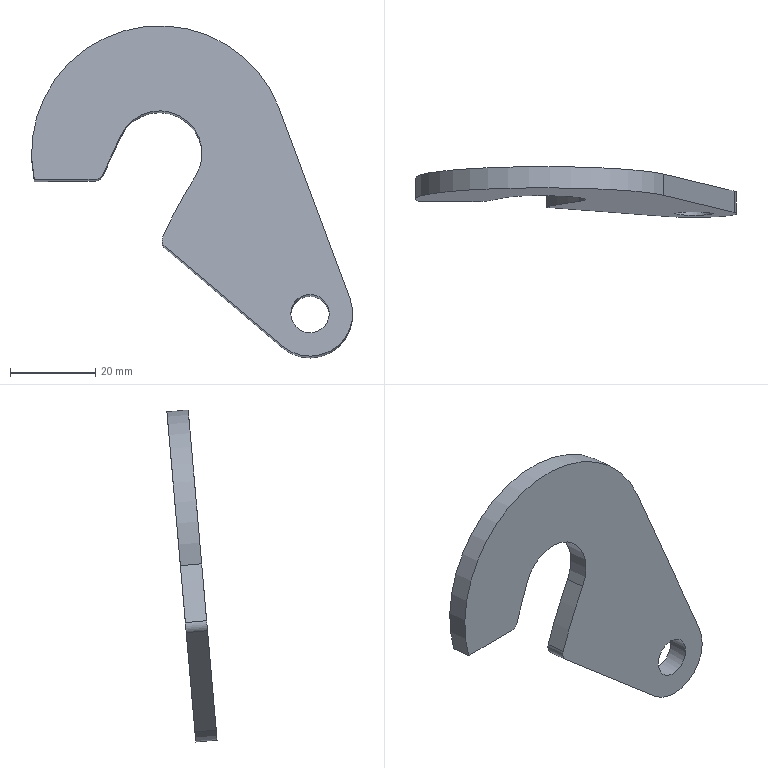Component | NX | HOOK_BAFFLE | 1 solid | 13 faces | box 75.29 x 11.76 x 77.87 mm | volume 13326 mm3 | cylinder 7 | plane 6 | commonest cylinder face diameters 20 x2 4 x2 60 x1 254.505 x1 9 x1
STEP:
#1=CARTESIAN_POINT('',(0.,0.,0.));
#2=DIRECTION('',(0.,0.,1.));
#3=DIRECTION('',(1.,0.,0.));
#4=AXIS2_PLACEMENT_3D('',#1,#2,#3);
#5=CARTESIAN_POINT('',(364.754,540.035,-52.402));
#6=VERTEX_POINT('',#5);
#7=CARTESIAN_POINT('',(380.609,541.002,-41.353));
#8=VERTEX_POINT('',#7);
#9=CARTESIAN_POINT('',(371.23,540.7,-44.811));
#10=DIRECTION('',(0.,-0.9962,0.08716));
#11=DIRECTION('',(-1.,-0.0006658,-0.00761));
#12=AXIS2_PLACEMENT_3D('',#9,#10,#11);
#13=CIRCLE('',#12,10.);
#14=CARTESIAN_POINT('',(371.23,545.681,-45.247));
#15=DIRECTION('',(0.,-0.9962,0.08716));
#16=DIRECTION('',(-0.00764,0.08715,0.9962));
#17=AXIS2_PLACEMENT_3D('',#14,#15,#16);
#18=CYLINDRICAL_SURFACE('',#17,10.);
#19=CARTESIAN_POINT('',(1.571,5.));
#20=DIRECTION('',(1.,-0.));
#21=VECTOR('',#20,1.);
#22=LINE('',#19,#21);
#23=(GEOMETRIC_REPRESENTATION_CONTEXT(2)PARAMETRIC_REPRESENTATION_CONTEXT()REPRESENTATION_CONTEXT('',''));
#24=DEFINITIONAL_REPRESENTATION('',(#22),#23);
#25=PCURVE('',#18,#24);
#26=CARTESIAN_POINT('',(371.23,540.7,-44.811));
#27=DIRECTION('',(0.,-0.9962,0.08716));
#28=DIRECTION('',(-0.00764,0.08715,0.9962));
#29=AXIS2_PLACEMENT_3D('',#26,#27,#28);
#30=PLANE('',#29);
#31=CARTESIAN_POINT('',(0.,0.));
#32=DIRECTION('',(0.,1.));
#33=AXIS2_PLACEMENT_2D('',#31,#32);
#34=CIRCLE('',#33,10.);
#35=(GEOMETRIC_REPRESENTATION_CONTEXT(2)PARAMETRIC_REPRESENTATION_CONTEXT()REPRESENTATION_CONTEXT('',''));
#36=DEFINITIONAL_REPRESENTATION('',(#34),#35);
#37=PCURVE('',#30,#36);
#38=SURFACE_CURVE('',#13,(#25,#37),.PCURVE_S1.);
#39=EDGE_CURVE('',#6,#8,#38,.T.);
#40=ORIENTED_EDGE('',*,*,#39,.F.);
#41=CARTESIAN_POINT('',(364.754,545.016,-52.838));
#42=VERTEX_POINT('',#41);
#43=CARTESIAN_POINT('',(364.754,545.016,-52.838));
#44=DIRECTION('',(0.,-0.9962,0.08716));
#45=VECTOR('',#44,1.);
#46=LINE('',#43,#45);
#47=CARTESIAN_POINT('',(2.43,-0.));
#48=DIRECTION('',(0.,1.));
#49=VECTOR('',#48,1.);
#50=LINE('',#47,#49);
#51=(GEOMETRIC_REPRESENTATION_CONTEXT(2)PARAMETRIC_REPRESENTATION_CONTEXT()REPRESENTATION_CONTEXT('',''));
#52=DEFINITIONAL_REPRESENTATION('',(#50),#51);
#53=PCURVE('',#18,#52);
#54=CARTESIAN_POINT('',(336.102,547.139,-28.578));
#55=DIRECTION('',(-0.6476,-0.06641,-0.7591));
#56=DIRECTION('',(-0.762,0.05644,0.6451));
#57=AXIS2_PLACEMENT_3D('',#54,#55,#56);
#58=PLANE('',#57);
#59=CARTESIAN_POINT('',(-37.603,0.));
#60=DIRECTION('',(0.,-1.));
#61=VECTOR('',#60,1.);
#62=LINE('',#59,#61);
#63=(GEOMETRIC_REPRESENTATION_CONTEXT(2)PARAMETRIC_REPRESENTATION_CONTEXT()REPRESENTATION_CONTEXT('',''));
#64=DEFINITIONAL_REPRESENTATION('',(#62),#63);
#65=PCURVE('',#58,#64);
#66=SURFACE_CURVE('',#46,(#53,#65),.PCURVE_S1.);
#67=EDGE_CURVE('',#42,#6,#66,.T.);
#68=ORIENTED_EDGE('',*,*,#67,.F.);
#69=CARTESIAN_POINT('',(380.609,545.983,-41.789));
#70=VERTEX_POINT('',#69);
#71=CARTESIAN_POINT('',(371.23,545.681,-45.247));
#72=DIRECTION('',(0.,-0.9962,0.08716));
#73=DIRECTION('',(-1.,-0.0006658,-0.00761));
#74=AXIS2_PLACEMENT_3D('',#71,#72,#73);
#75=CIRCLE('',#74,10.);
#76=CARTESIAN_POINT('',(1.571,0.));
#77=DIRECTION('',(1.,-0.));
#78=VECTOR('',#77,1.);
#79=LINE('',#76,#78);
#80=(GEOMETRIC_REPRESENTATION_CONTEXT(2)PARAMETRIC_REPRESENTATION_CONTEXT()REPRESENTATION_CONTEXT('',''));
#81=DEFINITIONAL_REPRESENTATION('',(#79),#80);
#82=PCURVE('',#18,#81);
#83=CARTESIAN_POINT('',(371.23,545.681,-45.247));
#84=DIRECTION('',(0.,-0.9962,0.08716));
#85=DIRECTION('',(-0.00764,0.08715,0.9962));
#86=AXIS2_PLACEMENT_3D('',#83,#84,#85);
#87=PLANE('',#86);
#88=CARTESIAN_POINT('',(0.,0.));
#89=DIRECTION('',(0.,1.));
#90=AXIS2_PLACEMENT_2D('',#88,#89);
#91=CIRCLE('',#90,10.);
#92=(GEOMETRIC_REPRESENTATION_CONTEXT(2)PARAMETRIC_REPRESENTATION_CONTEXT()REPRESENTATION_CONTEXT('',''));
#93=DEFINITIONAL_REPRESENTATION('',(#91),#92);
#94=PCURVE('',#87,#93);
#95=SURFACE_CURVE('',#75,(#82,#94),.PCURVE_S1.);
#96=EDGE_CURVE('',#42,#70,#95,.T.);
#97=ORIENTED_EDGE('',*,*,#96,.T.);
#98=CARTESIAN_POINT('',(380.609,545.983,-41.789));
#99=DIRECTION('',(0.,-0.9962,0.08716));
#100=VECTOR('',#99,1.);
#101=LINE('',#98,#100);
#102=CARTESIAN_POINT('',(5.059,-0.));
#103=DIRECTION('',(-0.,1.));
#104=VECTOR('',#103,1.);
#105=LINE('',#102,#104);
#106=(GEOMETRIC_REPRESENTATION_CONTEXT(2)PARAMETRIC_REPRESENTATION_CONTEXT()REPRESENTATION_CONTEXT('',''));
#107=DEFINITIONAL_REPRESENTATION('',(#105),#106);
#108=PCURVE('',#18,#107);
#109=CARTESIAN_POINT('',(380.609,545.983,-41.789));
#110=DIRECTION('',(0.9378,0.03025,0.3458));
#111=DIRECTION('',(0.3471,-0.08174,-0.9343));
#112=AXIS2_PLACEMENT_3D('',#109,#110,#111);
#113=PLANE('',#112);
#114=CARTESIAN_POINT('',(-0.,-0.));
#115=DIRECTION('',(-0.,-1.));
#116=VECTOR('',#115,1.);
#117=LINE('',#114,#116);
#118=(GEOMETRIC_REPRESENTATION_CONTEXT(2)PARAMETRIC_REPRESENTATION_CONTEXT()REPRESENTATION_CONTEXT('',''));
#119=DEFINITIONAL_REPRESENTATION('',(#117),#118);
#120=PCURVE('',#113,#119);
#121=SURFACE_CURVE('',#101,(#108,#120),.PCURVE_S1.);
#122=EDGE_CURVE('',#70,#8,#121,.T.);
#123=ORIENTED_EDGE('',*,*,#122,.T.);
#124=EDGE_LOOP('',(#40,#68,#97,#123));
#125=FACE_BOUND('',#124,.T.);
#126=ADVANCED_FACE('',(#125),#18,.T.);
#127=CARTESIAN_POINT('',(364.076,544.896,3.15));
#128=VERTEX_POINT('',#127);
#129=CARTESIAN_POINT('',(380.609,541.002,-41.353));
#130=DIRECTION('',(-0.3471,0.08174,0.9343));
#131=VECTOR('',#130,1.);
#132=LINE('',#129,#131);
#133=CARTESIAN_POINT('',(0.,-5.));
#134=DIRECTION('',(-1.,0.));
#135=VECTOR('',#134,1.);
#136=LINE('',#133,#135);
#137=(GEOMETRIC_REPRESENTATION_CONTEXT(2)PARAMETRIC_REPRESENTATION_CONTEXT()REPRESENTATION_CONTEXT('',''));
#138=DEFINITIONAL_REPRESENTATION('',(#136),#137);
#139=PCURVE('',#113,#138);
#140=CARTESIAN_POINT('',(3.399,-9.405));
#141=DIRECTION('',(0.9405,0.3399));
#142=VECTOR('',#141,1.);
#143=LINE('',#140,#142);
#144=(GEOMETRIC_REPRESENTATION_CONTEXT(2)PARAMETRIC_REPRESENTATION_CONTEXT()REPRESENTATION_CONTEXT('',''));
#145=DEFINITIONAL_REPRESENTATION('',(#143),#144);
#146=PCURVE('',#30,#145);
#147=SURFACE_CURVE('',#132,(#139,#146),.PCURVE_S1.);
#148=EDGE_CURVE('',#8,#128,#147,.T.);
#149=ORIENTED_EDGE('',*,*,#148,.F.);
#150=ORIENTED_EDGE('',*,*,#122,.F.);
#151=CARTESIAN_POINT('',(364.076,549.877,2.714));
#152=VERTEX_POINT('',#151);
#153=CARTESIAN_POINT('',(380.609,545.983,-41.789));
#154=DIRECTION('',(-0.3471,0.08174,0.9343));
#155=VECTOR('',#154,1.);
#156=LINE('',#153,#155);
#157=CARTESIAN_POINT('',(0.,0.));
#158=DIRECTION('',(-1.,0.));
#159=VECTOR('',#158,1.);
#160=LINE('',#157,#159);
#161=(GEOMETRIC_REPRESENTATION_CONTEXT(2)PARAMETRIC_REPRESENTATION_CONTEXT()REPRESENTATION_CONTEXT('',''));
#162=DEFINITIONAL_REPRESENTATION('',(#160),#161);
#163=PCURVE('',#113,#162);
#164=CARTESIAN_POINT('',(3.399,-9.405));
#165=DIRECTION('',(0.9405,0.3399));
#166=VECTOR('',#165,1.);
#167=LINE('',#164,#166);
#168=(GEOMETRIC_REPRESENTATION_CONTEXT(2)PARAMETRIC_REPRESENTATION_CONTEXT()REPRESENTATION_CONTEXT('',''));
#169=DEFINITIONAL_REPRESENTATION('',(#167),#168);
#170=PCURVE('',#87,#169);
#171=SURFACE_CURVE('',#156,(#163,#170),.PCURVE_S1.);
#172=EDGE_CURVE('',#70,#152,#171,.T.);
#173=ORIENTED_EDGE('',*,*,#172,.T.);
#174=CARTESIAN_POINT('',(364.076,549.877,2.714));
#175=DIRECTION('',(0.,-0.9962,0.08716));
#176=VECTOR('',#175,1.);
#177=LINE('',#174,#176);
#178=CARTESIAN_POINT('',(-47.634,0.));
#179=DIRECTION('',(-0.,-1.));
#180=VECTOR('',#179,1.);
#181=LINE('',#178,#180);
#182=(GEOMETRIC_REPRESENTATION_CONTEXT(2)PARAMETRIC_REPRESENTATION_CONTEXT()REPRESENTATION_CONTEXT('',''));
#183=DEFINITIONAL_REPRESENTATION('',(#181),#182);
#184=PCURVE('',#113,#183);
#185=CARTESIAN_POINT('',(335.941,548.969,-7.659));
#186=DIRECTION('',(0.,-0.9962,0.08716));
#187=DIRECTION('',(-0.00764,0.08715,0.9962));
#188=AXIS2_PLACEMENT_3D('',#185,#186,#187);
#189=CYLINDRICAL_SURFACE('',#188,30.);
#190=CARTESIAN_POINT('',(-1.224,-0.));
#191=DIRECTION('',(0.,1.));
#192=VECTOR('',#191,1.);
#193=LINE('',#190,#192);
#194=(GEOMETRIC_REPRESENTATION_CONTEXT(2)PARAMETRIC_REPRESENTATION_CONTEXT()REPRESENTATION_CONTEXT('',''));
#195=DEFINITIONAL_REPRESENTATION('',(#193),#194);
#196=PCURVE('',#189,#195);
#197=SURFACE_CURVE('',#177,(#184,#196),.PCURVE_S1.);
#198=EDGE_CURVE('',#152,#128,#197,.T.);
#199=ORIENTED_EDGE('',*,*,#198,.T.);
#200=EDGE_LOOP('',(#149,#150,#173,#199));
#201=FACE_BOUND('',#200,.T.);
#202=ADVANCED_FACE('',(#201),#113,.T.);
#203=CARTESIAN_POINT('',(306.594,543.446,-13.424));
#204=VERTEX_POINT('',#203);
#205=CARTESIAN_POINT('',(335.941,543.988,-7.223));
#206=DIRECTION('',(0.,-0.9962,0.08716));
#207=DIRECTION('',(-1.,-0.0006658,-0.00761));
#208=AXIS2_PLACEMENT_3D('',#205,#206,#207);
#209=CIRCLE('',#208,30.);
#210=CARTESIAN_POINT('',(-4.712,5.));
#211=DIRECTION('',(1.,0.));
#212=VECTOR('',#211,1.);
#213=LINE('',#210,#212);
#214=(GEOMETRIC_REPRESENTATION_CONTEXT(2)PARAMETRIC_REPRESENTATION_CONTEXT()REPRESENTATION_CONTEXT('',''));
#215=DEFINITIONAL_REPRESENTATION('',(#213),#214);
#216=PCURVE('',#189,#215);
#217=CARTESIAN_POINT('',(38.,35.));
#218=DIRECTION('',(0.,1.));
#219=AXIS2_PLACEMENT_2D('',#217,#218);
#220=CIRCLE('',#219,30.);
#221=(GEOMETRIC_REPRESENTATION_CONTEXT(2)PARAMETRIC_REPRESENTATION_CONTEXT()REPRESENTATION_CONTEXT('',''));
#222=DEFINITIONAL_REPRESENTATION('',(#220),#221);
#223=PCURVE('',#30,#222);
#224=SURFACE_CURVE('',#209,(#216,#223),.PCURVE_S1.);
#225=EDGE_CURVE('',#128,#204,#224,.T.);
#226=ORIENTED_EDGE('',*,*,#225,.F.);
#227=ORIENTED_EDGE('',*,*,#198,.F.);
#228=CARTESIAN_POINT('',(306.594,548.427,-13.86));
#229=VERTEX_POINT('',#228);
#230=CARTESIAN_POINT('',(335.941,548.969,-7.659));
#231=DIRECTION('',(0.,-0.9962,0.08716));
#232=DIRECTION('',(-1.,-0.0006658,-0.00761));
#233=AXIS2_PLACEMENT_3D('',#230,#231,#232);
#234=CIRCLE('',#233,30.);
#235=CARTESIAN_POINT('',(-4.712,0.));
#236=DIRECTION('',(1.,-0.));
#237=VECTOR('',#236,1.);
#238=LINE('',#235,#237);
#239=(GEOMETRIC_REPRESENTATION_CONTEXT(2)PARAMETRIC_REPRESENTATION_CONTEXT()REPRESENTATION_CONTEXT('',''));
#240=DEFINITIONAL_REPRESENTATION('',(#238),#239);
#241=PCURVE('',#189,#240);
#242=CARTESIAN_POINT('',(38.,35.));
#243=DIRECTION('',(0.,1.));
#244=AXIS2_PLACEMENT_2D('',#242,#243);
#245=CIRCLE('',#244,30.);
#246=(GEOMETRIC_REPRESENTATION_CONTEXT(2)PARAMETRIC_REPRESENTATION_CONTEXT()REPRESENTATION_CONTEXT('',''));
#247=DEFINITIONAL_REPRESENTATION('',(#245),#246);
#248=PCURVE('',#87,#247);
#249=SURFACE_CURVE('',#234,(#241,#248),.PCURVE_S1.);
#250=EDGE_CURVE('',#152,#229,#249,.T.);
#251=ORIENTED_EDGE('',*,*,#250,.T.);
#252=CARTESIAN_POINT('',(306.594,548.427,-13.86));
#253=DIRECTION('',(0.,-0.9962,0.08716));
#254=VECTOR('',#253,1.);
#255=LINE('',#252,#254);
#256=CARTESIAN_POINT('',(1.772,-0.));
#257=DIRECTION('',(0.,1.));
#258=VECTOR('',#257,1.);
#259=LINE('',#256,#258);
#260=(GEOMETRIC_REPRESENTATION_CONTEXT(2)PARAMETRIC_REPRESENTATION_CONTEXT()REPRESENTATION_CONTEXT('',''));
#261=DEFINITIONAL_REPRESENTATION('',(#259),#260);
#262=PCURVE('',#189,#261);
#263=CARTESIAN_POINT('',(306.594,548.427,-13.86));
#264=DIRECTION('',(0.00764,-0.08715,-0.9962));
#265=DIRECTION('',(-0.,-0.9962,0.08716));
#266=AXIS2_PLACEMENT_3D('',#263,#264,#265);
#267=PLANE('',#266);
#268=CARTESIAN_POINT('',(0.,0.));
#269=DIRECTION('',(1.,0.));
#270=VECTOR('',#269,1.);
#271=LINE('',#268,#270);
#272=(GEOMETRIC_REPRESENTATION_CONTEXT(2)PARAMETRIC_REPRESENTATION_CONTEXT()REPRESENTATION_CONTEXT('',''));
#273=DEFINITIONAL_REPRESENTATION('',(#271),#272);
#274=PCURVE('',#267,#273);
#275=SURFACE_CURVE('',#255,(#262,#274),.PCURVE_S1.);
#276=EDGE_CURVE('',#229,#204,#275,.T.);
#277=ORIENTED_EDGE('',*,*,#276,.T.);
#278=EDGE_LOOP('',(#226,#227,#251,#277));
#279=FACE_BOUND('',#278,.T.);
#280=ADVANCED_FACE('',(#279),#189,.T.);
#281=CARTESIAN_POINT('',(320.846,548.436,-13.751));
#282=VERTEX_POINT('',#281);
#283=CARTESIAN_POINT('',(306.594,548.427,-13.86));
#284=DIRECTION('',(1.,0.0006658,0.00761));
#285=VECTOR('',#284,1.);
#286=LINE('',#283,#285);
#287=CARTESIAN_POINT('',(0.,0.));
#288=DIRECTION('',(-0.,-1.));
#289=VECTOR('',#288,1.);
#290=LINE('',#287,#289);
#291=(GEOMETRIC_REPRESENTATION_CONTEXT(2)PARAMETRIC_REPRESENTATION_CONTEXT()REPRESENTATION_CONTEXT('',''));
#292=DEFINITIONAL_REPRESENTATION('',(#290),#291);
#293=PCURVE('',#267,#292);
#294=CARTESIAN_POINT('',(32.,64.394));
#295=DIRECTION('',(-0.,-1.));
#296=VECTOR('',#295,1.);
#297=LINE('',#294,#296);
#298=(GEOMETRIC_REPRESENTATION_CONTEXT(2)PARAMETRIC_REPRESENTATION_CONTEXT()REPRESENTATION_CONTEXT('',''));
#299=DEFINITIONAL_REPRESENTATION('',(#297),#298);
#300=PCURVE('',#87,#299);
#301=SURFACE_CURVE('',#286,(#293,#300),.PCURVE_S1.);
#302=EDGE_CURVE('',#229,#282,#301,.T.);
#303=ORIENTED_EDGE('',*,*,#302,.T.);
#304=CARTESIAN_POINT('',(320.846,543.455,-13.315));
#305=VERTEX_POINT('',#304);
#306=CARTESIAN_POINT('',(320.846,548.436,-13.751));
#307=DIRECTION('',(0.,-0.9962,0.08716));
#308=VECTOR('',#307,1.);
#309=LINE('',#306,#308);
#310=CARTESIAN_POINT('',(0.,-14.252));
#311=DIRECTION('',(1.,0.));
#312=VECTOR('',#311,1.);
#313=LINE('',#310,#312);
#314=(GEOMETRIC_REPRESENTATION_CONTEXT(2)PARAMETRIC_REPRESENTATION_CONTEXT()REPRESENTATION_CONTEXT('',''));
#315=DEFINITIONAL_REPRESENTATION('',(#313),#314);
#316=PCURVE('',#267,#315);
#317=CARTESIAN_POINT('',(320.83,548.61,-11.759));
#318=DIRECTION('',(0.,-0.9962,0.08716));
#319=DIRECTION('',(-0.00764,0.08715,0.9962));
#320=AXIS2_PLACEMENT_3D('',#317,#318,#319);
#321=CYLINDRICAL_SURFACE('',#320,2.);
#322=CARTESIAN_POINT('',(3.142,0.));
#323=DIRECTION('',(0.,1.));
#324=VECTOR('',#323,1.);
#325=LINE('',#322,#324);
#326=(GEOMETRIC_REPRESENTATION_CONTEXT(2)PARAMETRIC_REPRESENTATION_CONTEXT()REPRESENTATION_CONTEXT('',''));
#327=DEFINITIONAL_REPRESENTATION('',(#325),#326);
#328=PCURVE('',#321,#327);
#329=SURFACE_CURVE('',#309,(#316,#328),.PCURVE_S1.);
#330=EDGE_CURVE('',#282,#305,#329,.T.);
#331=ORIENTED_EDGE('',*,*,#330,.T.);
#332=CARTESIAN_POINT('',(306.594,543.446,-13.424));
#333=DIRECTION('',(1.,0.0006658,0.00761));
#334=VECTOR('',#333,1.);
#335=LINE('',#332,#334);
#336=CARTESIAN_POINT('',(5.,-0.));
#337=DIRECTION('',(-0.,-1.));
#338=VECTOR('',#337,1.);
#339=LINE('',#336,#338);
#340=(GEOMETRIC_REPRESENTATION_CONTEXT(2)PARAMETRIC_REPRESENTATION_CONTEXT()REPRESENTATION_CONTEXT('',''));
#341=DEFINITIONAL_REPRESENTATION('',(#339),#340);
#342=PCURVE('',#267,#341);
#343=CARTESIAN_POINT('',(32.,64.394));
#344=DIRECTION('',(-0.,-1.));
#345=VECTOR('',#344,1.);
#346=LINE('',#343,#345);
#347=(GEOMETRIC_REPRESENTATION_CONTEXT(2)PARAMETRIC_REPRESENTATION_CONTEXT()REPRESENTATION_CONTEXT('',''));
#348=DEFINITIONAL_REPRESENTATION('',(#346),#347);
#349=PCURVE('',#30,#348);
#350=SURFACE_CURVE('',#335,(#342,#349),.PCURVE_S1.);
#351=EDGE_CURVE('',#204,#305,#350,.T.);
#352=ORIENTED_EDGE('',*,*,#351,.F.);
#353=ORIENTED_EDGE('',*,*,#276,.F.);
#354=EDGE_LOOP('',(#303,#331,#352,#353));
#355=FACE_BOUND('',#354,.T.);
#356=ADVANCED_FACE('',(#355),#267,.T.);
#357=CARTESIAN_POINT('',(322.647,543.556,-12.157));
#358=VERTEX_POINT('',#357);
#359=CARTESIAN_POINT('',(326.86,544.353,-3.053));
#360=VERTEX_POINT('',#359);
#361=CARTESIAN_POINT('',(322.115,543.456,-13.306));
#362=DIRECTION('',(0.4186,0.07915,0.9047));
#363=VECTOR('',#362,1.);
#364=LINE('',#361,#363);
#365=CARTESIAN_POINT('',(322.115,548.437,-13.741));
#366=DIRECTION('',(0.9082,-0.03649,-0.417));
#367=DIRECTION('',(-0.4186,-0.07915,-0.9047));
#368=AXIS2_PLACEMENT_3D('',#365,#366,#367);
#369=PLANE('',#368);
#370=CARTESIAN_POINT('',(0.,-5.));
#371=DIRECTION('',(-1.,-0.));
#372=VECTOR('',#371,1.);
#373=LINE('',#370,#372);
#374=(GEOMETRIC_REPRESENTATION_CONTEXT(2)PARAMETRIC_REPRESENTATION_CONTEXT()REPRESENTATION_CONTEXT('',''));
#375=DEFINITIONAL_REPRESENTATION('',(#373),#374);
#376=PCURVE('',#369,#375);
#377=CARTESIAN_POINT('',(32.,48.872));
#378=DIRECTION('',(0.9049,-0.4256));
#379=VECTOR('',#378,1.);
#380=LINE('',#377,#379);
#381=(GEOMETRIC_REPRESENTATION_CONTEXT(2)PARAMETRIC_REPRESENTATION_CONTEXT()REPRESENTATION_CONTEXT('',''));
#382=DEFINITIONAL_REPRESENTATION('',(#380),#381);
#383=PCURVE('',#30,#382);
#384=SURFACE_CURVE('',#364,(#376,#383),.PCURVE_S1.);
#385=EDGE_CURVE('',#358,#360,#384,.T.);
#386=ORIENTED_EDGE('',*,*,#385,.F.);
#387=CARTESIAN_POINT('',(322.647,548.537,-12.593));
#388=VERTEX_POINT('',#387);
#389=CARTESIAN_POINT('',(322.647,548.537,-12.593));
#390=DIRECTION('',(0.,0.9962,-0.08716));
#391=VECTOR('',#390,1.);
#392=LINE('',#389,#391);
#393=CARTESIAN_POINT('',(-1.27,-0.));
#394=DIRECTION('',(-0.,1.));
#395=VECTOR('',#394,1.);
#396=LINE('',#393,#395);
#397=(GEOMETRIC_REPRESENTATION_CONTEXT(2)PARAMETRIC_REPRESENTATION_CONTEXT()REPRESENTATION_CONTEXT('',''));
#398=DEFINITIONAL_REPRESENTATION('',(#396),#397);
#399=PCURVE('',#369,#398);
#400=CARTESIAN_POINT('',(4.273,0.));
#401=DIRECTION('',(0.,-1.));
#402=VECTOR('',#401,1.);
#403=LINE('',#400,#402);
#404=(GEOMETRIC_REPRESENTATION_CONTEXT(2)PARAMETRIC_REPRESENTATION_CONTEXT()REPRESENTATION_CONTEXT('',''));
#405=DEFINITIONAL_REPRESENTATION('',(#403),#404);
#406=PCURVE('',#321,#405);
#407=SURFACE_CURVE('',#392,(#399,#406),.PCURVE_S1.);
#408=EDGE_CURVE('',#358,#388,#407,.T.);
#409=ORIENTED_EDGE('',*,*,#408,.T.);
#410=CARTESIAN_POINT('',(326.86,549.334,-3.488));
#411=VERTEX_POINT('',#410);
#412=CARTESIAN_POINT('',(322.115,548.437,-13.741));
#413=DIRECTION('',(0.4186,0.07915,0.9047));
#414=VECTOR('',#413,1.);
#415=LINE('',#412,#414);
#416=CARTESIAN_POINT('',(0.,0.));
#417=DIRECTION('',(-1.,-0.));
#418=VECTOR('',#417,1.);
#419=LINE('',#416,#418);
#420=(GEOMETRIC_REPRESENTATION_CONTEXT(2)PARAMETRIC_REPRESENTATION_CONTEXT()REPRESENTATION_CONTEXT('',''));
#421=DEFINITIONAL_REPRESENTATION('',(#419),#420);
#422=PCURVE('',#369,#421);
#423=CARTESIAN_POINT('',(32.,48.872));
#424=DIRECTION('',(0.9049,-0.4256));
#425=VECTOR('',#424,1.);
#426=LINE('',#423,#425);
#427=(GEOMETRIC_REPRESENTATION_CONTEXT(2)PARAMETRIC_REPRESENTATION_CONTEXT()REPRESENTATION_CONTEXT('',''));
#428=DEFINITIONAL_REPRESENTATION('',(#426),#427);
#429=PCURVE('',#87,#428);
#430=SURFACE_CURVE('',#415,(#422,#429),.PCURVE_S1.);
#431=EDGE_CURVE('',#388,#411,#430,.T.);
#432=ORIENTED_EDGE('',*,*,#431,.T.);
#433=CARTESIAN_POINT('',(326.86,549.334,-3.488));
#434=DIRECTION('',(0.,-0.9962,0.08716));
#435=VECTOR('',#434,1.);
#436=LINE('',#433,#435);
#437=CARTESIAN_POINT('',(-11.333,-0.));
#438=DIRECTION('',(0.,-1.));
#439=VECTOR('',#438,1.);
#440=LINE('',#437,#439);
#441=(GEOMETRIC_REPRESENTATION_CONTEXT(2)PARAMETRIC_REPRESENTATION_CONTEXT()REPRESENTATION_CONTEXT('',''));
#442=DEFINITIONAL_REPRESENTATION('',(#440),#441);
#443=PCURVE('',#369,#442);
#444=CARTESIAN_POINT('',(335.941,548.969,-7.659));
#445=DIRECTION('',(0.,-0.9962,0.08716));
#446=DIRECTION('',(-0.00764,0.08715,0.9962));
#447=AXIS2_PLACEMENT_3D('',#444,#445,#446);
#448=CYLINDRICAL_SURFACE('',#447,10.);
#449=CARTESIAN_POINT('',(7.414,-0.));
#450=DIRECTION('',(0.,1.));
#451=VECTOR('',#450,1.);
#452=LINE('',#449,#451);
#453=(GEOMETRIC_REPRESENTATION_CONTEXT(2)PARAMETRIC_REPRESENTATION_CONTEXT()REPRESENTATION_CONTEXT('',''));
#454=DEFINITIONAL_REPRESENTATION('',(#452),#453);
#455=PCURVE('',#448,#454);
#456=SURFACE_CURVE('',#436,(#443,#455),.PCURVE_S1.);
#457=EDGE_CURVE('',#411,#360,#456,.T.);
#458=ORIENTED_EDGE('',*,*,#457,.T.);
#459=EDGE_LOOP('',(#386,#409,#432,#458));
#460=FACE_BOUND('',#459,.T.);
#461=ADVANCED_FACE('',(#460),#369,.T.);
#462=CARTESIAN_POINT('',(344.428,548.508,-12.928));
#463=VERTEX_POINT('',#462);
#464=CARTESIAN_POINT('',(344.428,543.527,-12.492));
#465=VERTEX_POINT('',#464);
#466=CARTESIAN_POINT('',(344.428,548.508,-12.928));
#467=DIRECTION('',(0.,-0.9962,0.08716));
#468=VECTOR('',#467,1.);
#469=LINE('',#466,#468);
#470=CARTESIAN_POINT('',(4.147,-0.));
#471=DIRECTION('',(0.,1.));
#472=VECTOR('',#471,1.);
#473=LINE('',#470,#472);
#474=(GEOMETRIC_REPRESENTATION_CONTEXT(2)PARAMETRIC_REPRESENTATION_CONTEXT()REPRESENTATION_CONTEXT('',''));
#475=DEFINITIONAL_REPRESENTATION('',(#473),#474);
#476=PCURVE('',#448,#475);
#477=CARTESIAN_POINT('',(452.427,542.643,-79.972));
#478=DIRECTION('',(0.,-0.9962,0.08716));
#479=DIRECTION('',(-0.00764,0.08715,0.9962));
#480=AXIS2_PLACEMENT_3D('',#477,#478,#479);
#481=CYLINDRICAL_SURFACE('',#480,127.252);
#482=CARTESIAN_POINT('',(1.006,0.));
#483=DIRECTION('',(0.,1.));
#484=VECTOR('',#483,1.);
#485=LINE('',#482,#484);
#486=(GEOMETRIC_REPRESENTATION_CONTEXT(2)PARAMETRIC_REPRESENTATION_CONTEXT()REPRESENTATION_CONTEXT('',''));
#487=DEFINITIONAL_REPRESENTATION('',(#485),#486);
#488=PCURVE('',#481,#487);
#489=SURFACE_CURVE('',#469,(#476,#488),.PCURVE_S1.);
#490=EDGE_CURVE('',#463,#465,#489,.T.);
#491=ORIENTED_EDGE('',*,*,#490,.F.);
#492=CARTESIAN_POINT('',(335.941,548.969,-7.659));
#493=DIRECTION('',(-0.,0.9962,-0.08716));
#494=DIRECTION('',(-1.,-0.0006658,-0.00761));
#495=AXIS2_PLACEMENT_3D('',#492,#493,#494);
#496=CIRCLE('',#495,10.);
#497=CARTESIAN_POINT('',(7.854,-0.));
#498=DIRECTION('',(-1.,0.));
#499=VECTOR('',#498,1.);
#500=LINE('',#497,#499);
#501=(GEOMETRIC_REPRESENTATION_CONTEXT(2)PARAMETRIC_REPRESENTATION_CONTEXT()REPRESENTATION_CONTEXT('',''));
#502=DEFINITIONAL_REPRESENTATION('',(#500),#501);
#503=PCURVE('',#448,#502);
#504=CARTESIAN_POINT('',(38.,45.));
#505=CARTESIAN_POINT('',(55.321,45.));
#506=CARTESIAN_POINT('',(46.66,30.));
#507=CARTESIAN_POINT('',(38.,15.));
#508=CARTESIAN_POINT('',(29.34,30.));
#509=CARTESIAN_POINT('',(20.679,45.));
#510=CARTESIAN_POINT('',(38.,45.));
#511=(BOUNDED_CURVE()B_SPLINE_CURVE(2,(#504,#505,#506,#507,#508,#509,#510),.UNSPECIFIED.,.T.,.F.)B_SPLINE_CURVE_WITH_KNOTS((1,2,2,2,2,1),(-2.094,0.,2.094,4.189,6.283,8.378),.UNSPECIFIED.)CURVE()GEOMETRIC_REPRESENTATION_ITEM()RATIONAL_B_SPLINE_CURVE((1.,0.5,1.,0.5,1.,0.5,1.))REPRESENTATION_ITEM(''));
#512=(GEOMETRIC_REPRESENTATION_CONTEXT(2)PARAMETRIC_REPRESENTATION_CONTEXT()REPRESENTATION_CONTEXT('',''));
#513=DEFINITIONAL_REPRESENTATION('',(#511),#512);
#514=PCURVE('',#87,#513);
#515=SURFACE_CURVE('',#496,(#503,#514),.PCURVE_S1.);
#516=EDGE_CURVE('',#411,#463,#515,.T.);
#517=ORIENTED_EDGE('',*,*,#516,.F.);
#518=ORIENTED_EDGE('',*,*,#457,.T.);
#519=CARTESIAN_POINT('',(335.941,543.988,-7.223));
#520=DIRECTION('',(-0.,0.9962,-0.08716));
#521=DIRECTION('',(-1.,-0.0006658,-0.00761));
#522=AXIS2_PLACEMENT_3D('',#519,#520,#521);
#523=CIRCLE('',#522,10.);
#524=CARTESIAN_POINT('',(7.854,5.));
#525=DIRECTION('',(-1.,-0.));
#526=VECTOR('',#525,1.);
#527=LINE('',#524,#526);
#528=(GEOMETRIC_REPRESENTATION_CONTEXT(2)PARAMETRIC_REPRESENTATION_CONTEXT()REPRESENTATION_CONTEXT('',''));
#529=DEFINITIONAL_REPRESENTATION('',(#527),#528);
#530=PCURVE('',#448,#529);
#531=CARTESIAN_POINT('',(38.,45.));
#532=CARTESIAN_POINT('',(55.321,45.));
#533=CARTESIAN_POINT('',(46.66,30.));
#534=CARTESIAN_POINT('',(38.,15.));
#535=CARTESIAN_POINT('',(29.34,30.));
#536=CARTESIAN_POINT('',(20.679,45.));
#537=CARTESIAN_POINT('',(38.,45.));
#538=(BOUNDED_CURVE()B_SPLINE_CURVE(2,(#531,#532,#533,#534,#535,#536,#537),.UNSPECIFIED.,.T.,.F.)B_SPLINE_CURVE_WITH_KNOTS((1,2,2,2,2,1),(-2.094,0.,2.094,4.189,6.283,8.378),.UNSPECIFIED.)CURVE()GEOMETRIC_REPRESENTATION_ITEM()RATIONAL_B_SPLINE_CURVE((1.,0.5,1.,0.5,1.,0.5,1.))REPRESENTATION_ITEM(''));
#539=(GEOMETRIC_REPRESENTATION_CONTEXT(2)PARAMETRIC_REPRESENTATION_CONTEXT()REPRESENTATION_CONTEXT('',''));
#540=DEFINITIONAL_REPRESENTATION('',(#538),#539);
#541=PCURVE('',#30,#540);
#542=SURFACE_CURVE('',#523,(#530,#541),.PCURVE_S1.);
#543=EDGE_CURVE('',#360,#465,#542,.T.);
#544=ORIENTED_EDGE('',*,*,#543,.T.);
#545=EDGE_LOOP('',(#491,#517,#518,#544));
#546=FACE_BOUND('',#545,.F.);
#547=ADVANCED_FACE('',(#546),#448,.F.);
#548=CARTESIAN_POINT('',(336.724,547.259,-27.201));
#549=VERTEX_POINT('',#548);
#550=CARTESIAN_POINT('',(452.427,542.643,-79.972));
#551=DIRECTION('',(0.,-0.9962,0.08716));
#552=DIRECTION('',(-1.,-0.0006658,-0.00761));
#553=AXIS2_PLACEMENT_3D('',#550,#551,#552);
#554=CIRCLE('',#553,127.252);
#555=CARTESIAN_POINT('',(-4.712,0.));
#556=DIRECTION('',(1.,-0.));
#557=VECTOR('',#556,1.);
#558=LINE('',#555,#557);
#559=(GEOMETRIC_REPRESENTATION_CONTEXT(2)PARAMETRIC_REPRESENTATION_CONTEXT()REPRESENTATION_CONTEXT('',''));
#560=DEFINITIONAL_REPRESENTATION('',(#558),#559);
#561=PCURVE('',#481,#560);
#562=CARTESIAN_POINT('',(-35.477,-80.928));
#563=DIRECTION('',(0.,1.));
#564=AXIS2_PLACEMENT_2D('',#562,#563);
#565=CIRCLE('',#564,127.252);
#566=(GEOMETRIC_REPRESENTATION_CONTEXT(2)PARAMETRIC_REPRESENTATION_CONTEXT()REPRESENTATION_CONTEXT('',''));
#567=DEFINITIONAL_REPRESENTATION('',(#565),#566);
#568=PCURVE('',#87,#567);
#569=SURFACE_CURVE('',#554,(#561,#568),.PCURVE_S1.);
#570=EDGE_CURVE('',#463,#549,#569,.T.);
#571=ORIENTED_EDGE('',*,*,#570,.T.);
#572=CARTESIAN_POINT('',(336.724,542.278,-26.765));
#573=VERTEX_POINT('',#572);
#574=CARTESIAN_POINT('',(336.724,547.259,-27.201));
#575=DIRECTION('',(0.,-0.9962,0.08716));
#576=VECTOR('',#575,1.);
#577=LINE('',#574,#576);
#578=CARTESIAN_POINT('',(1.134,-0.));
#579=DIRECTION('',(0.,1.));
#580=VECTOR('',#579,1.);
#581=LINE('',#578,#580);
#582=(GEOMETRIC_REPRESENTATION_CONTEXT(2)PARAMETRIC_REPRESENTATION_CONTEXT()REPRESENTATION_CONTEXT('',''));
#583=DEFINITIONAL_REPRESENTATION('',(#581),#582);
#584=PCURVE('',#481,#583);
#585=CARTESIAN_POINT('',(338.543,547.187,-28.031));
#586=DIRECTION('',(0.,-0.9962,0.08716));
#587=DIRECTION('',(-0.00764,0.08715,0.9962));
#588=AXIS2_PLACEMENT_3D('',#585,#586,#587);
#589=CYLINDRICAL_SURFACE('',#588,2.);
#590=CARTESIAN_POINT('',(1.134,0.));
#591=DIRECTION('',(0.,1.));
#592=VECTOR('',#591,1.);
#593=LINE('',#590,#592);
#594=(GEOMETRIC_REPRESENTATION_CONTEXT(2)PARAMETRIC_REPRESENTATION_CONTEXT()REPRESENTATION_CONTEXT('',''));
#595=DEFINITIONAL_REPRESENTATION('',(#593),#594);
#596=PCURVE('',#589,#595);
#597=SURFACE_CURVE('',#577,(#584,#596),.PCURVE_S1.);
#598=EDGE_CURVE('',#549,#573,#597,.T.);
#599=ORIENTED_EDGE('',*,*,#598,.T.);
#600=CARTESIAN_POINT('',(452.427,537.662,-79.536));
#601=DIRECTION('',(0.,-0.9962,0.08716));
#602=DIRECTION('',(-1.,-0.0006658,-0.00761));
#603=AXIS2_PLACEMENT_3D('',#600,#601,#602);
#604=CIRCLE('',#603,127.252);
#605=CARTESIAN_POINT('',(-4.712,5.));
#606=DIRECTION('',(1.,0.));
#607=VECTOR('',#606,1.);
#608=LINE('',#605,#607);
#609=(GEOMETRIC_REPRESENTATION_CONTEXT(2)PARAMETRIC_REPRESENTATION_CONTEXT()REPRESENTATION_CONTEXT('',''));
#610=DEFINITIONAL_REPRESENTATION('',(#608),#609);
#611=PCURVE('',#481,#610);
#612=CARTESIAN_POINT('',(-35.477,-80.928));
#613=DIRECTION('',(0.,1.));
#614=AXIS2_PLACEMENT_2D('',#612,#613);
#615=CIRCLE('',#614,127.252);
#616=(GEOMETRIC_REPRESENTATION_CONTEXT(2)PARAMETRIC_REPRESENTATION_CONTEXT()REPRESENTATION_CONTEXT('',''));
#617=DEFINITIONAL_REPRESENTATION('',(#615),#616);
#618=PCURVE('',#30,#617);
#619=SURFACE_CURVE('',#604,(#611,#618),.PCURVE_S1.);
#620=EDGE_CURVE('',#465,#573,#619,.T.);
#621=ORIENTED_EDGE('',*,*,#620,.F.);
#622=ORIENTED_EDGE('',*,*,#490,.F.);
#623=EDGE_LOOP('',(#571,#599,#621,#622));
#624=FACE_BOUND('',#623,.T.);
#625=ADVANCED_FACE('',(#624),#481,.T.);
#626=CARTESIAN_POINT('',(337.248,542.073,-29.113));
#627=VERTEX_POINT('',#626);
#628=CARTESIAN_POINT('',(336.102,542.158,-28.143));
#629=DIRECTION('',(0.762,-0.05644,-0.6451));
#630=VECTOR('',#629,1.);
#631=LINE('',#628,#630);
#632=CARTESIAN_POINT('',(0.,-5.));
#633=DIRECTION('',(-1.,0.));
#634=VECTOR('',#633,1.);
#635=LINE('',#632,#634);
#636=(GEOMETRIC_REPRESENTATION_CONTEXT(2)PARAMETRIC_REPRESENTATION_CONTEXT()REPRESENTATION_CONTEXT('',''));
#637=DEFINITIONAL_REPRESENTATION('',(#635),#636);
#638=PCURVE('',#58,#637);
#639=CARTESIAN_POINT('',(17.,35.));
#640=DIRECTION('',(-0.6534,-0.757));
#641=VECTOR('',#640,1.);
#642=LINE('',#639,#641);
#643=(GEOMETRIC_REPRESENTATION_CONTEXT(2)PARAMETRIC_REPRESENTATION_CONTEXT()REPRESENTATION_CONTEXT('',''));
#644=DEFINITIONAL_REPRESENTATION('',(#642),#643);
#645=PCURVE('',#30,#644);
#646=SURFACE_CURVE('',#631,(#638,#645),.PCURVE_S1.);
#647=EDGE_CURVE('',#627,#6,#646,.T.);
#648=ORIENTED_EDGE('',*,*,#647,.F.);
#649=CARTESIAN_POINT('',(337.248,547.054,-29.549));
#650=VERTEX_POINT('',#649);
#651=CARTESIAN_POINT('',(337.248,547.054,-29.549));
#652=DIRECTION('',(0.,0.9962,-0.08716));
#653=VECTOR('',#652,1.);
#654=LINE('',#651,#653);
#655=CARTESIAN_POINT('',(-1.504,0.));
#656=DIRECTION('',(-0.,1.));
#657=VECTOR('',#656,1.);
#658=LINE('',#655,#657);
#659=(GEOMETRIC_REPRESENTATION_CONTEXT(2)PARAMETRIC_REPRESENTATION_CONTEXT()REPRESENTATION_CONTEXT('',''));
#660=DEFINITIONAL_REPRESENTATION('',(#658),#659);
#661=PCURVE('',#58,#660);
#662=CARTESIAN_POINT('',(2.43,0.));
#663=DIRECTION('',(0.,-1.));
#664=VECTOR('',#663,1.);
#665=LINE('',#662,#664);
#666=(GEOMETRIC_REPRESENTATION_CONTEXT(2)PARAMETRIC_REPRESENTATION_CONTEXT()REPRESENTATION_CONTEXT('',''));
#667=DEFINITIONAL_REPRESENTATION('',(#665),#666);
#668=PCURVE('',#589,#667);
#669=SURFACE_CURVE('',#654,(#661,#668),.PCURVE_S1.);
#670=EDGE_CURVE('',#627,#650,#669,.T.);
#671=ORIENTED_EDGE('',*,*,#670,.T.);
#672=CARTESIAN_POINT('',(336.102,547.139,-28.578));
#673=DIRECTION('',(0.762,-0.05644,-0.6451));
#674=VECTOR('',#673,1.);
#675=LINE('',#672,#674);
#676=CARTESIAN_POINT('',(0.,0.));
#677=DIRECTION('',(-1.,0.));
#678=VECTOR('',#677,1.);
#679=LINE('',#676,#678);
#680=(GEOMETRIC_REPRESENTATION_CONTEXT(2)PARAMETRIC_REPRESENTATION_CONTEXT()REPRESENTATION_CONTEXT('',''));
#681=DEFINITIONAL_REPRESENTATION('',(#679),#680);
#682=PCURVE('',#58,#681);
#683=CARTESIAN_POINT('',(17.,35.));
#684=DIRECTION('',(-0.6534,-0.757));
#685=VECTOR('',#684,1.);
#686=LINE('',#683,#685);
#687=(GEOMETRIC_REPRESENTATION_CONTEXT(2)PARAMETRIC_REPRESENTATION_CONTEXT()REPRESENTATION_CONTEXT('',''));
#688=DEFINITIONAL_REPRESENTATION('',(#686),#687);
#689=PCURVE('',#87,#688);
#690=SURFACE_CURVE('',#675,(#682,#689),.PCURVE_S1.);
#691=EDGE_CURVE('',#650,#42,#690,.T.);
#692=ORIENTED_EDGE('',*,*,#691,.T.);
#693=ORIENTED_EDGE('',*,*,#67,.T.);
#694=EDGE_LOOP('',(#648,#671,#692,#693));
#695=FACE_BOUND('',#694,.T.);
#696=ADVANCED_FACE('',(#695),#58,.T.);
#697=CARTESIAN_POINT('',(371.196,546.073,-40.764));
#698=VERTEX_POINT('',#697);
#699=CARTESIAN_POINT('',(371.23,545.681,-45.247));
#700=DIRECTION('',(0.,0.9962,-0.08716));
#701=DIRECTION('',(-0.00764,0.08715,0.9962));
#702=AXIS2_PLACEMENT_3D('',#699,#700,#701);
#703=CIRCLE('',#702,4.5);
#704=CARTESIAN_POINT('',(4.5,-0.));
#705=CARTESIAN_POINT('',(4.5,-7.794));
#706=CARTESIAN_POINT('',(-2.25,-3.897));
#707=CARTESIAN_POINT('',(-9.,0.));
#708=CARTESIAN_POINT('',(-2.25,3.897));
#709=CARTESIAN_POINT('',(4.5,7.794));
#710=CARTESIAN_POINT('',(4.5,-0.));
#711=(BOUNDED_CURVE()B_SPLINE_CURVE(2,(#704,#705,#706,#707,#708,#709,#710),.UNSPECIFIED.,.T.,.F.)B_SPLINE_CURVE_WITH_KNOTS((1,2,2,2,2,1),(-2.094,0.,2.094,4.189,6.283,8.378),.UNSPECIFIED.)CURVE()GEOMETRIC_REPRESENTATION_ITEM()RATIONAL_B_SPLINE_CURVE((1.,0.5,1.,0.5,1.,0.5,1.))REPRESENTATION_ITEM(''));
#712=(GEOMETRIC_REPRESENTATION_CONTEXT(2)PARAMETRIC_REPRESENTATION_CONTEXT()REPRESENTATION_CONTEXT('',''));
#713=DEFINITIONAL_REPRESENTATION('',(#711),#712);
#714=PCURVE('',#87,#713);
#715=CARTESIAN_POINT('',(371.23,580.547,-48.297));
#716=DIRECTION('',(0.,-0.9962,0.08716));
#717=DIRECTION('',(-0.00764,0.08715,0.9962));
#718=AXIS2_PLACEMENT_3D('',#715,#716,#717);
#719=CYLINDRICAL_SURFACE('',#718,4.5);
#720=CARTESIAN_POINT('',(6.283,35.));
#721=DIRECTION('',(-1.,0.));
#722=VECTOR('',#721,1.);
#723=LINE('',#720,#722);
#724=(GEOMETRIC_REPRESENTATION_CONTEXT(2)PARAMETRIC_REPRESENTATION_CONTEXT()REPRESENTATION_CONTEXT('',''));
#725=DEFINITIONAL_REPRESENTATION('',(#723),#724);
#726=PCURVE('',#719,#725);
#727=SURFACE_CURVE('',#703,(#714,#726),.PCURVE_S1.);
#728=EDGE_CURVE('',#698,#698,#727,.T.);
#729=ORIENTED_EDGE('',*,*,#728,.F.);
#730=EDGE_LOOP('',(#729));
#731=FACE_BOUND('',#730,.T.);
#732=ORIENTED_EDGE('',*,*,#431,.F.);
#733=CARTESIAN_POINT('',(320.83,548.61,-11.759));
#734=DIRECTION('',(0.,0.9962,-0.08716));
#735=DIRECTION('',(-0.00764,0.08715,0.9962));
#736=AXIS2_PLACEMENT_3D('',#733,#734,#735);
#737=CIRCLE('',#736,2.);
#738=CARTESIAN_POINT('',(36.,50.142));
#739=CARTESIAN_POINT('',(36.,46.678));
#740=CARTESIAN_POINT('',(33.,48.41));
#741=CARTESIAN_POINT('',(30.,50.142));
#742=CARTESIAN_POINT('',(33.,51.874));
#743=CARTESIAN_POINT('',(36.,53.606));
#744=CARTESIAN_POINT('',(36.,50.142));
#745=(BOUNDED_CURVE()B_SPLINE_CURVE(2,(#738,#739,#740,#741,#742,#743,#744),.UNSPECIFIED.,.T.,.F.)B_SPLINE_CURVE_WITH_KNOTS((1,2,2,2,2,1),(-2.094,0.,2.094,4.189,6.283,8.378),.UNSPECIFIED.)CURVE()GEOMETRIC_REPRESENTATION_ITEM()RATIONAL_B_SPLINE_CURVE((1.,0.5,1.,0.5,1.,0.5,1.))REPRESENTATION_ITEM(''));
#746=(GEOMETRIC_REPRESENTATION_CONTEXT(2)PARAMETRIC_REPRESENTATION_CONTEXT()REPRESENTATION_CONTEXT('',''));
#747=DEFINITIONAL_REPRESENTATION('',(#745),#746);
#748=PCURVE('',#87,#747);
#749=CARTESIAN_POINT('',(6.283,0.));
#750=DIRECTION('',(-1.,0.));
#751=VECTOR('',#750,1.);
#752=LINE('',#749,#751);
#753=(GEOMETRIC_REPRESENTATION_CONTEXT(2)PARAMETRIC_REPRESENTATION_CONTEXT()REPRESENTATION_CONTEXT('',''));
#754=DEFINITIONAL_REPRESENTATION('',(#752),#753);
#755=PCURVE('',#321,#754);
#756=SURFACE_CURVE('',#737,(#748,#755),.PCURVE_S1.);
#757=EDGE_CURVE('',#388,#282,#756,.T.);
#758=ORIENTED_EDGE('',*,*,#757,.T.);
#759=ORIENTED_EDGE('',*,*,#302,.F.);
#760=ORIENTED_EDGE('',*,*,#250,.F.);
#761=ORIENTED_EDGE('',*,*,#172,.F.);
#762=ORIENTED_EDGE('',*,*,#96,.F.);
#763=ORIENTED_EDGE('',*,*,#691,.F.);
#764=CARTESIAN_POINT('',(338.543,547.187,-28.031));
#765=DIRECTION('',(0.,0.9962,-0.08716));
#766=DIRECTION('',(-0.00764,0.08715,0.9962));
#767=AXIS2_PLACEMENT_3D('',#764,#765,#766);
#768=CIRCLE('',#767,2.);
#769=CARTESIAN_POINT('',(19.531,32.554));
#770=CARTESIAN_POINT('',(19.531,29.09));
#771=CARTESIAN_POINT('',(16.531,30.822));
#772=CARTESIAN_POINT('',(13.531,32.554));
#773=CARTESIAN_POINT('',(16.531,34.286));
#774=CARTESIAN_POINT('',(19.531,36.019));
#775=CARTESIAN_POINT('',(19.531,32.554));
#776=(BOUNDED_CURVE()B_SPLINE_CURVE(2,(#769,#770,#771,#772,#773,#774,#775),.UNSPECIFIED.,.T.,.F.)B_SPLINE_CURVE_WITH_KNOTS((1,2,2,2,2,1),(-2.094,0.,2.094,4.189,6.283,8.378),.UNSPECIFIED.)CURVE()GEOMETRIC_REPRESENTATION_ITEM()RATIONAL_B_SPLINE_CURVE((1.,0.5,1.,0.5,1.,0.5,1.))REPRESENTATION_ITEM(''));
#777=(GEOMETRIC_REPRESENTATION_CONTEXT(2)PARAMETRIC_REPRESENTATION_CONTEXT()REPRESENTATION_CONTEXT('',''));
#778=DEFINITIONAL_REPRESENTATION('',(#776),#777);
#779=PCURVE('',#87,#778);
#780=CARTESIAN_POINT('',(6.283,0.));
#781=DIRECTION('',(-1.,-0.));
#782=VECTOR('',#781,1.);
#783=LINE('',#780,#782);
#784=(GEOMETRIC_REPRESENTATION_CONTEXT(2)PARAMETRIC_REPRESENTATION_CONTEXT()REPRESENTATION_CONTEXT('',''));
#785=DEFINITIONAL_REPRESENTATION('',(#783),#784);
#786=PCURVE('',#589,#785);
#787=SURFACE_CURVE('',#768,(#779,#786),.PCURVE_S1.);
#788=EDGE_CURVE('',#650,#549,#787,.T.);
#789=ORIENTED_EDGE('',*,*,#788,.T.);
#790=ORIENTED_EDGE('',*,*,#570,.F.);
#791=ORIENTED_EDGE('',*,*,#516,.F.);
#792=EDGE_LOOP('',(#732,#758,#759,#760,#761,#762,#763,#789,#790,#791));
#793=FACE_BOUND('',#792,.T.);
#794=ADVANCED_FACE('',(#731,#793),#87,.F.);
#795=CARTESIAN_POINT('',(366.731,540.697,-44.845));
#796=VERTEX_POINT('',#795);
#797=CARTESIAN_POINT('',(371.196,541.092,-40.328));
#798=VERTEX_POINT('',#797);
#799=CARTESIAN_POINT('',(371.23,540.7,-44.811));
#800=DIRECTION('',(0.,0.9962,-0.08716));
#801=DIRECTION('',(-1.,-0.0006658,-0.00761));
#802=AXIS2_PLACEMENT_3D('',#799,#800,#801);
#803=CIRCLE('',#802,4.5);
#804=CARTESIAN_POINT('',(0.,4.5));
#805=CARTESIAN_POINT('',(7.794,4.5));
#806=CARTESIAN_POINT('',(3.897,-2.25));
#807=CARTESIAN_POINT('',(-0.,-9.));
#808=CARTESIAN_POINT('',(-3.897,-2.25));
#809=CARTESIAN_POINT('',(-7.794,4.5));
#810=CARTESIAN_POINT('',(0.,4.5));
#811=(BOUNDED_CURVE()B_SPLINE_CURVE(2,(#804,#805,#806,#807,#808,#809,#810),.UNSPECIFIED.,.T.,.F.)B_SPLINE_CURVE_WITH_KNOTS((1,2,2,2,2,1),(-2.094,0.,2.094,4.189,6.283,8.378),.UNSPECIFIED.)CURVE()GEOMETRIC_REPRESENTATION_ITEM()RATIONAL_B_SPLINE_CURVE((1.,0.5,1.,0.5,1.,0.5,1.))REPRESENTATION_ITEM(''));
#812=(GEOMETRIC_REPRESENTATION_CONTEXT(2)PARAMETRIC_REPRESENTATION_CONTEXT()REPRESENTATION_CONTEXT('',''));
#813=DEFINITIONAL_REPRESENTATION('',(#811),#812);
#814=PCURVE('',#30,#813);
#815=CARTESIAN_POINT('',(1.571,40.));
#816=DIRECTION('',(-1.,0.));
#817=VECTOR('',#816,1.);
#818=LINE('',#815,#817);
#819=(GEOMETRIC_REPRESENTATION_CONTEXT(2)PARAMETRIC_REPRESENTATION_CONTEXT()REPRESENTATION_CONTEXT('',''));
#820=DEFINITIONAL_REPRESENTATION('',(#818),#819);
#821=PCURVE('',#719,#820);
#822=SURFACE_CURVE('',#803,(#814,#821),.PCURVE_S1.);
#823=EDGE_CURVE('',#796,#798,#822,.T.);
#824=ORIENTED_EDGE('',*,*,#823,.T.);
#825=CARTESIAN_POINT('',(371.23,540.7,-44.811));
#826=DIRECTION('',(0.,0.9962,-0.08716));
#827=DIRECTION('',(-1.,-0.0006658,-0.00761));
#828=AXIS2_PLACEMENT_3D('',#825,#826,#827);
#829=CIRCLE('',#828,4.5);
#830=CARTESIAN_POINT('',(0.,4.5));
#831=CARTESIAN_POINT('',(7.794,4.5));
#832=CARTESIAN_POINT('',(3.897,-2.25));
#833=CARTESIAN_POINT('',(-0.,-9.));
#834=CARTESIAN_POINT('',(-3.897,-2.25));
#835=CARTESIAN_POINT('',(-7.794,4.5));
#836=CARTESIAN_POINT('',(0.,4.5));
#837=(BOUNDED_CURVE()B_SPLINE_CURVE(2,(#830,#831,#832,#833,#834,#835,#836),.UNSPECIFIED.,.T.,.F.)B_SPLINE_CURVE_WITH_KNOTS((1,2,2,2,2,1),(-2.094,0.,2.094,4.189,6.283,8.378),.UNSPECIFIED.)CURVE()GEOMETRIC_REPRESENTATION_ITEM()RATIONAL_B_SPLINE_CURVE((1.,0.5,1.,0.5,1.,0.5,1.))REPRESENTATION_ITEM(''));
#838=(GEOMETRIC_REPRESENTATION_CONTEXT(2)PARAMETRIC_REPRESENTATION_CONTEXT()REPRESENTATION_CONTEXT('',''));
#839=DEFINITIONAL_REPRESENTATION('',(#837),#838);
#840=PCURVE('',#30,#839);
#841=CARTESIAN_POINT('',(7.854,40.));
#842=DIRECTION('',(-1.,0.));
#843=VECTOR('',#842,1.);
#844=LINE('',#841,#843);
#845=(GEOMETRIC_REPRESENTATION_CONTEXT(2)PARAMETRIC_REPRESENTATION_CONTEXT()REPRESENTATION_CONTEXT('',''));
#846=DEFINITIONAL_REPRESENTATION('',(#844),#845);
#847=PCURVE('',#719,#846);
#848=SURFACE_CURVE('',#829,(#840,#847),.PCURVE_S1.);
#849=EDGE_CURVE('',#798,#796,#848,.T.);
#850=ORIENTED_EDGE('',*,*,#849,.T.);
#851=EDGE_LOOP('',(#824,#850));
#852=FACE_BOUND('',#851,.T.);
#853=ORIENTED_EDGE('',*,*,#351,.T.);
#854=CARTESIAN_POINT('',(320.83,543.629,-11.323));
#855=DIRECTION('',(0.,-0.9962,0.08716));
#856=DIRECTION('',(-0.00764,0.08715,0.9962));
#857=AXIS2_PLACEMENT_3D('',#854,#855,#856);
#858=CIRCLE('',#857,2.);
#859=CARTESIAN_POINT('',(34.,50.142));
#860=DIRECTION('',(1.,-0.));
#861=AXIS2_PLACEMENT_2D('',#859,#860);
#862=CIRCLE('',#861,2.);
#863=(GEOMETRIC_REPRESENTATION_CONTEXT(2)PARAMETRIC_REPRESENTATION_CONTEXT()REPRESENTATION_CONTEXT('',''));
#864=DEFINITIONAL_REPRESENTATION('',(#862),#863);
#865=PCURVE('',#30,#864);
#866=CARTESIAN_POINT('',(0.,5.));
#867=DIRECTION('',(1.,0.));
#868=VECTOR('',#867,1.);
#869=LINE('',#866,#868);
#870=(GEOMETRIC_REPRESENTATION_CONTEXT(2)PARAMETRIC_REPRESENTATION_CONTEXT()REPRESENTATION_CONTEXT('',''));
#871=DEFINITIONAL_REPRESENTATION('',(#869),#870);
#872=PCURVE('',#321,#871);
#873=SURFACE_CURVE('',#858,(#865,#872),.PCURVE_S1.);
#874=EDGE_CURVE('',#305,#358,#873,.T.);
#875=ORIENTED_EDGE('',*,*,#874,.T.);
#876=ORIENTED_EDGE('',*,*,#385,.T.);
#877=ORIENTED_EDGE('',*,*,#543,.T.);
#878=ORIENTED_EDGE('',*,*,#620,.T.);
#879=CARTESIAN_POINT('',(338.543,542.206,-27.595));
#880=DIRECTION('',(0.,-0.9962,0.08716));
#881=DIRECTION('',(-0.00764,0.08715,0.9962));
#882=AXIS2_PLACEMENT_3D('',#879,#880,#881);
#883=CIRCLE('',#882,2.);
#884=CARTESIAN_POINT('',(17.531,32.554));
#885=DIRECTION('',(1.,-0.));
#886=AXIS2_PLACEMENT_2D('',#884,#885);
#887=CIRCLE('',#886,2.);
#888=(GEOMETRIC_REPRESENTATION_CONTEXT(2)PARAMETRIC_REPRESENTATION_CONTEXT()REPRESENTATION_CONTEXT('',''));
#889=DEFINITIONAL_REPRESENTATION('',(#887),#888);
#890=PCURVE('',#30,#889);
#891=CARTESIAN_POINT('',(0.,5.));
#892=DIRECTION('',(1.,0.));
#893=VECTOR('',#892,1.);
#894=LINE('',#891,#893);
#895=(GEOMETRIC_REPRESENTATION_CONTEXT(2)PARAMETRIC_REPRESENTATION_CONTEXT()REPRESENTATION_CONTEXT('',''));
#896=DEFINITIONAL_REPRESENTATION('',(#894),#895);
#897=PCURVE('',#589,#896);
#898=SURFACE_CURVE('',#883,(#890,#897),.PCURVE_S1.);
#899=EDGE_CURVE('',#573,#627,#898,.T.);
#900=ORIENTED_EDGE('',*,*,#899,.T.);
#901=ORIENTED_EDGE('',*,*,#647,.T.);
#902=ORIENTED_EDGE('',*,*,#39,.T.);
#903=ORIENTED_EDGE('',*,*,#148,.T.);
#904=ORIENTED_EDGE('',*,*,#225,.T.);
#905=EDGE_LOOP('',(#853,#875,#876,#877,#878,#900,#901,#902,#903,#904));
#906=FACE_BOUND('',#905,.T.);
#907=ADVANCED_FACE('',(#852,#906),#30,.T.);
#908=ORIENTED_EDGE('',*,*,#823,.T.);
#909=CARTESIAN_POINT('',(371.196,546.073,-40.764));
#910=CARTESIAN_POINT('',(371.196,541.092,-40.328));
#911=B_SPLINE_CURVE_WITH_KNOTS('',1,(#909,#910),.UNSPECIFIED.,.F.,.F.,(2,2),(35.,40.),.PIECEWISE_BEZIER_KNOTS.);
#912=CARTESIAN_POINT('',(0.,0.));
#913=DIRECTION('',(0.,1.));
#914=VECTOR('',#913,1.);
#915=LINE('',#912,#914);
#916=(GEOMETRIC_REPRESENTATION_CONTEXT(2)PARAMETRIC_REPRESENTATION_CONTEXT()REPRESENTATION_CONTEXT('',''));
#917=DEFINITIONAL_REPRESENTATION('',(#915),#916);
#918=PCURVE('',#719,#917);
#919=CARTESIAN_POINT('',(6.283,0.));
#920=DIRECTION('',(0.,1.));
#921=VECTOR('',#920,1.);
#922=LINE('',#919,#921);
#923=(GEOMETRIC_REPRESENTATION_CONTEXT(2)PARAMETRIC_REPRESENTATION_CONTEXT()REPRESENTATION_CONTEXT('',''));
#924=DEFINITIONAL_REPRESENTATION('',(#922),#923);
#925=PCURVE('',#719,#924);
#926=SEAM_CURVE('',#911,(#918,#925),.PCURVE_S1.);
#927=EDGE_CURVE('',#698,#798,#926,.T.);
#928=ORIENTED_EDGE('',*,*,#927,.F.);
#929=ORIENTED_EDGE('',*,*,#728,.F.);
#930=ORIENTED_EDGE('',*,*,#927,.T.);
#931=ORIENTED_EDGE('',*,*,#849,.T.);
#932=EDGE_LOOP('',(#908,#928,#929,#930,#931));
#933=FACE_BOUND('',#932,.F.);
#934=ADVANCED_FACE('',(#933),#719,.F.);
#935=ORIENTED_EDGE('',*,*,#788,.F.);
#936=ORIENTED_EDGE('',*,*,#670,.F.);
#937=ORIENTED_EDGE('',*,*,#899,.F.);
#938=ORIENTED_EDGE('',*,*,#598,.F.);
#939=EDGE_LOOP('',(#935,#936,#937,#938));
#940=FACE_BOUND('',#939,.T.);
#941=ADVANCED_FACE('',(#940),#589,.T.);
#942=ORIENTED_EDGE('',*,*,#757,.F.);
#943=ORIENTED_EDGE('',*,*,#408,.F.);
#944=ORIENTED_EDGE('',*,*,#874,.F.);
#945=ORIENTED_EDGE('',*,*,#330,.F.);
#946=EDGE_LOOP('',(#942,#943,#944,#945));
#947=FACE_BOUND('',#946,.T.);
#948=ADVANCED_FACE('',(#947),#321,.T.);
#949=CLOSED_SHELL('',(#126,#202,#280,#356,#461,#547,#625,#696,#794,#907,#934,#941,#948));
#950=MANIFOLD_SOLID_BREP('',#949);
#951=(LENGTH_UNIT()NAMED_UNIT(*)SI_UNIT(.MILLI.,.METRE.));
#952=UNCERTAINTY_MEASURE_WITH_UNIT(LENGTH_MEASURE(0.000001),#951,'','');
#953=(NAMED_UNIT(*)PLANE_ANGLE_UNIT()SI_UNIT($,.RADIAN.));
#954=(NAMED_UNIT(*)SI_UNIT($,.STERADIAN.)SOLID_ANGLE_UNIT());
#955=(GEOMETRIC_REPRESENTATION_CONTEXT(3)GLOBAL_UNCERTAINTY_ASSIGNED_CONTEXT((#952))GLOBAL_UNIT_ASSIGNED_CONTEXT((#951,#953,#954))REPRESENTATION_CONTEXT('',''));
#956=ADVANCED_BREP_SHAPE_REPRESENTATION('',(#4,#950),#955);